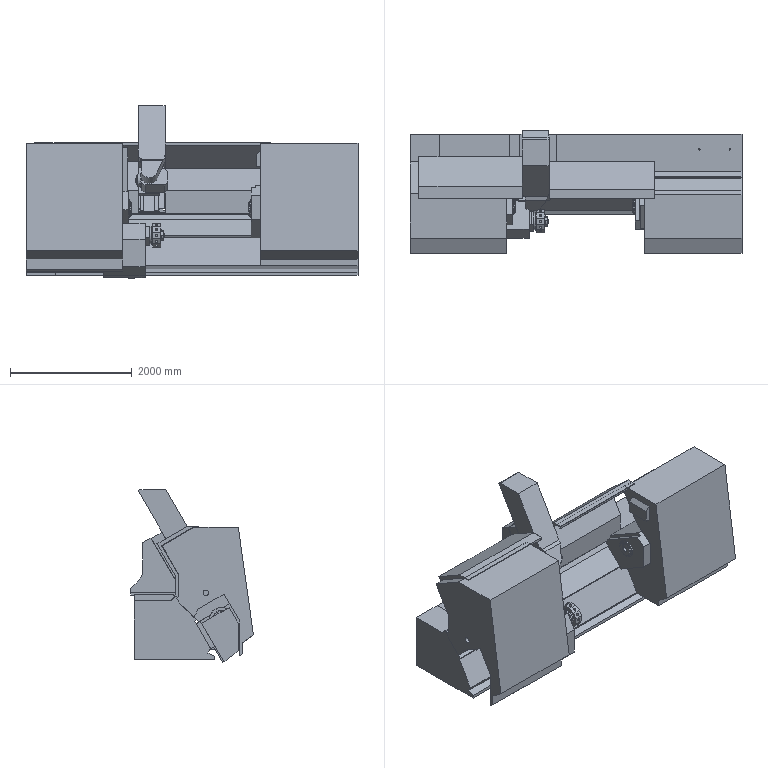Assembly | NX | mm | 20 component files | 21 solids | 1107 faces | box 5449 x 2015.31 x 2834.56 mm | volume 11701829959 mm3 | plane 863 | cylinder 149 | cone 93 | torus 2 | commonest cylinder face diameters 55.4 x40 54 x20 40 x12 495 x8 184 x4 154 x4 20 x3 270 x3
Bill of materials:
unnamed part 1 | 1 |  | Thin flat annular disc with a large central through-hole and one small through-hole near the outer rim.
unnamed part 2 | 1 |  | Cylinder with a thin, slightly larger-diameter flange at one end. The flange has a small rectangular notch in its rim.
unnamed part 3 | 1 |  | Prismatic block with chamfered corners, giving a roughly octagonal profile, with stepped coaxial cylindrical bosses projecting from one end and shallow circular recesses on the side faces.
unnamed part 4 | 1 |  | Flat rectangular slab with a narrow rectangular tongue running along one face and a matching rectangular groove along the opposite face.
unnamed part 5 | 1 |  | Solid block with a pentagonal cross-section (one corner bevelled) and a small rectangular tab protruding from one face.
unnamed part 6 | 1 |  | Square-section bar stepping down at a shoulder to a narrower tip section with a rounded end and an angled flank.
unnamed part 7 | 1 |  | Long straight extrusion with a constant, irregular polygonal cross-section: flat top and one flat vertical side, a stepped angled face on the other side, and small lips or ridges along the edges.
unnamed part 8 | 1 |  | Plain solid round rod with flat ends and a uniform diameter.
unnamed part 9 | 1 |  | Flat rectangular plate with two parallel raised rectangular ribs across its top face and an angled step along one bottom edge.
unnamed part 10 | 1 |  | Circular disc base with a ring of evenly spaced upright tabs around its perimeter. Each tab has a semicircular cutout at its top, and small inward-pointing tabs sit between them. A small slender post or pin feature is set off-center on the base.
unnamed part 11 | 1 |  | Thick ten-sided (decagonal) body with radial round holes through its flat side faces. One face has a raised circular rim or ring groove; the other face carries a stepped coaxial boss with a hex-shaped section.
unnamed part 12 | 1 |  | Prismatic part whose cross-section has a long sloped face, a vertical back face, and a filleted transition into a short horizontal foot. Two shallow longitudinal grooves run along the sloped face, and small rectangular tabs sit at the ends.
unnamed part 13 | 1 |  | Elongated prismatic block with an angled/chamfered lower end, two small rectangular notches along one top edge, a shallow circular recess or boss outline on one face, and a slender cylindrical pin protruding from that face.
unnamed part 14 | 1 |  | Short cylindrical disc on a slightly larger, thicker base that has four radial rectangular lugs or tabs. The base outline is stepped.
unnamed part 15 | 1 |  | Thin flat annular ring (washer-like) with a large central hole and one small through hole near the outer edge. A radial line on one face suggests a split or seam.
unnamed part 16 | 1 |  | Long, constant-section, thin-wall profile with several bends: a short horizontal top lip with a downturned flange, a long inclined segment, a second inclined segment, and a vertical leg ending in a small hooked/clip detail.
unnamed part 17 | 1 |  | Elongated prismatic bar with an irregular polygonal (pentagon/hexagon-like) cross-section and a small round axial hole on one end face. A short cylindrical stub or counterbore feature appears at one end.
unnamed part 18 | 1 |  | Long, constant-section, thin-wall bent profile very similar to unnamed part 16: top lip with downturned flange, inclined segments, vertical leg with small hooked end, and short stepped regions near one end.
unnamed part 19 | 1 |  | Solid block with an irregular polygonal end profile, including an inclined back face and a notched recess in one face. Small mounting pads with round holes, counterbore-like features and rectangular slots sit in the notch region.
unnamed part 20 | 1 |  | Solid prismatic block with an irregular polygonal end profile that has a V/stepped notch in one side, plus a small rectangular tab protruding from one end face.
Mates:
1. touch align | Sim15_Hauptspindelseite 1 face | Sim15_Maschinenbett 1 face
2. touch align | Sim15_Hauptspindelseite 1 face | Sim15_Maschinenbett 1 face
3. touch align | Sim15_Gegenspindel 1 face | Sim15_Maschinenbett 1 face
4. touch align | Sim15_Gegenspindel 1 edge | Sim15_Maschinenbett 1 edge
5. touch align | Sim15_Gegenspindelseite 1 face | Sim15_Gegenspindel 1 face
6. distance | Sim15_Gegenspindelseite 1 face | Sim15_Hauptspindelseite 1 face
7. touch align | Sim15_Gegenspindelseite 1 face | Sim15_Gegenspindel 1 face
8. touch align | Sim15_Z2_Schlitten 1 face | Sim15_Maschinenbett 1 face
9. touch align | Sim15_Z2_Schlitten 1 edge | Sim15_Maschinenbett 1 edge
10. touch align | Sim15_X2_Schlitten 1 face | Sim15_Z2_Schlitten 1 face
11. touch align | Sim15_X2_Schlitten 1 face | Sim15_Z2_Schlitten 1 face
12. distance | Sim15_X2_Schlitten 1 face | Sim15_C4_axis 1
13. touch align | Sim15_Rev_Scheibe_Aufnahme 1 face | Sim15_X2_Schlitten 1 face
14. parallel | Sim15_Rev_Scheibe_Aufnahme 1 edge | Sim15_X2_Schlitten 1 edge
15. parallel | Sim15_Rev_Scheibe_Aufnahme 1 face | Sim15_X2_Schlitten 1 face
16. distance | Sim15_Rev_Scheibe_Aufnahme 1 face | Sim15_X2_Schlitten 1 face
17. distance | Sim15_Rev_Scheibe_Aufnahme 1 face | Sim15_X2_Schlitten 1 face
18. touch align | Sim15_Rev_Scheibe 1 face | Sim15_Rev_Scheibe_Aufnahme 1 face
19. touch align | Sim15_Rev_Scheibe 1 edge | Sim15_Rev_Scheibe_Aufnahme 1 edge
20. angle | Sim15_Rev_Scheibe 1 face | Sim15_X2_Schlitten 1 face
21. distance | Sim15_Rev_Scheibe 1 | assembly datumaxis
22. touch align | Sim15_Z1_Schlitten 1 face | Sim15_Maschinenbett 1 face
23. touch align | Sim15_Z1_Schlitten 1 face | Sim15_Maschinenbett 1 face
24. touch align | Sim15_Abdeckung_oben_rechts 1 face | Sim15_Maschinenbett 1 face
25. touch align | Sim15_Abdeckung_oben_rechts 1 face | Sim15_Maschinenbett 1 face
26. touch align | Sim15_Abdeckung_oben_rechts 1 face | Sim15_B1_Achse_Deckel 1 face
27. touch align | Sim15_Abedeckung_oben_links_neu 1 face | Sim15_Maschinenbett 1 face
28. touch align | Sim15_Abedeckung_oben_links_neu 1 face | Sim15_Maschinenbett 1 face
29. touch align | Sim15_Abedeckung_oben_links_neu 1 face | Sim15_B1_Achse_Deckel 1 face
30. parallel | Sim15_B1_Achse 1 | Sim15_X1_Schlitten 1 face
31. touch align | Sim15_B1_Achse 1 | Sim15_X1_Schlitten 1 face
32. touch align | Sim15_B1_Achse 1 | Sim15_X1_Schlitten 1 face
33. touch align | Sim15_C1_Achse 1 face | Sim15_B1_Achse 1
34. touch align | Sim15_C1_Achse 1 face | Sim15_B1_Achse 1
35. touch align | Sim15_C4_axis 1 | Sim15_Hauptspindelseite 1 face
36. touch align | Sim15_C4_axis 1 | Sim15_Hauptspindelseite 1 face
37. parallel | Sim15_C4_axis 1 | Sim15_Hauptspindelseite 1 face
38. touch align | Sim15_C3_axis 1 | Sim15_Gegenspindel 1 face
39. touch align | Sim15_C3_axis 1 | Sim15_Gegenspindel 1 face
40. parallel | Sim15_C3_axis 1 | Sim15_Hauptspindelseite 1 face
41. touch align | Sim15_B1_Achse_Deckel 1 face | Sim15_B1_Achse 1
42. parallel | Sim15_B1_Achse_Deckel 1 face | Sim15_X1_Schlitten 1 face
43. touch align | Sim15_B1_Achse_Deckel 1 face | Sim15_B1_Achse 1
44. touch align | Sim15_c_spindelanschlag_116 1 | Sim15_Gegenspindel 1 face
45. distance | Sim15_c_spindelanschlag_116 1 | Sim15_Gegenspindel 1 face
46. fix | Sim15_X1_Schlitten 1 component
47. fix | Sim15_Maschinenbett 1 component
48. distance | sim15_Magazin 1 | Sim15_Hauptspindelseite 1 face
49. touch align | sim15_Magazin 1 | Sim15_Hauptspindelseite 1 face